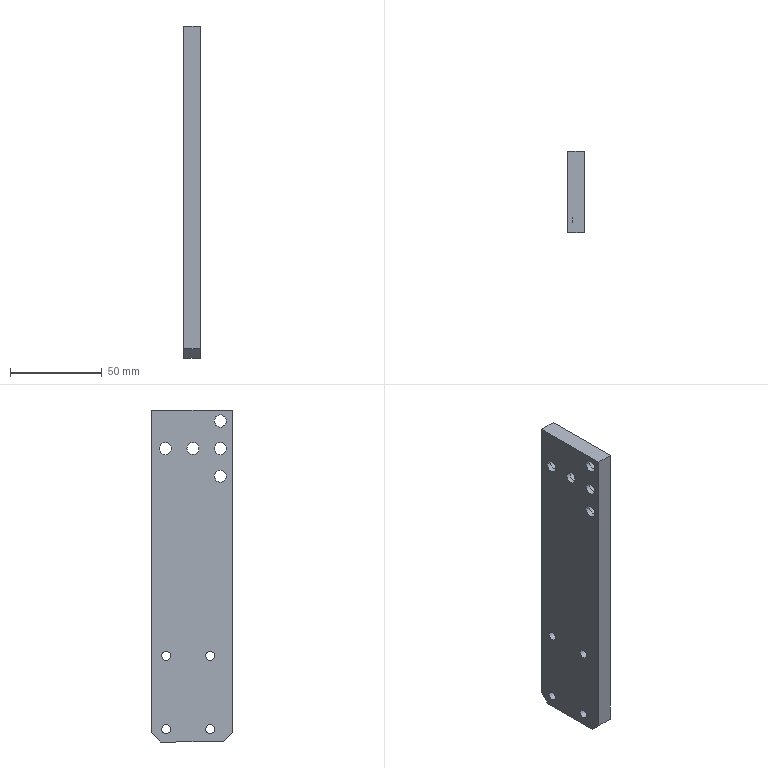Component | SolidWorks | 17081801-804-025A-1 | 1 solid | 41 faces | box 9 x 44 x 181 mm | volume 67258 mm3 | cylinder 28 | plane 13 | commonest cylinder face diameters 11 x10 6.6 x10 5 x8 | material AL6061
build123d program:
from build123d import *

# Parameters (mm, degrees)
SKETCH1_W                                       = 181
SKETCH1_H                                       = 44
BOSS_EXTRUDE1_DEPTH                             = 4.5
M6_TAPPED_HOLE1_D                               = 5
M6_TAPPED_HOLE1_DEPTH                           = 15
M6_TAPPED_HOLE1_TIP                             = 1.502
CHAMFER1_SIZE                                   = 5
M6_HEX_SOCKET_HEAD_CAP_SCREW_CBORE1_D           = 6.6
M6_HEX_SOCKET_HEAD_CAP_SCREW_CBORE1_DEPTH       = 15
M6_HEX_SOCKET_HEAD_CAP_SCREW_CBORE1_CBORE_D     = 11
M6_HEX_SOCKET_HEAD_CAP_SCREW_CBORE1_CBORE_DEPTH = 6.4
M6_HEX_SOCKET_HEAD_CAP_SCREW_CBORE1_TIP         = 1.983
M6_HEX_SOCKET_HEAD_CAP_SCREW_CBORE2_D           = 6.6
M6_HEX_SOCKET_HEAD_CAP_SCREW_CBORE2_DEPTH       = 15
M6_HEX_SOCKET_HEAD_CAP_SCREW_CBORE2_CBORE_D     = 11
M6_HEX_SOCKET_HEAD_CAP_SCREW_CBORE2_CBORE_DEPTH = 6.4
M6_HEX_SOCKET_HEAD_CAP_SCREW_CBORE2_TIP         = 1.983


with BuildPart() as part:
    # Sketch1 → Boss-Extrude1 (new, symmetric)
    with BuildSketch(Plane(origin=(0, 0, 0), x_dir=(1, 0, 0), z_dir=(0, 1, 0))):
        Rectangle(SKETCH1_W, SKETCH1_H)
    extrude(amount=BOSS_EXTRUDE1_DEPTH, both=True)

    # M6 Tapped Hole1
    with Locations(Plane(origin=(0, 4.5, 0), x_dir=(1, 0, 0), z_dir=(0, 1, 0))):
        with Locations((43.5, 10), (83.5, 10), (83.5, -14), (43.5, -14)):
            Hole(M6_TAPPED_HOLE1_D / 2, depth=M6_TAPPED_HOLE1_DEPTH)
            with Locations((0, 0, -(M6_TAPPED_HOLE1_DEPTH + M6_TAPPED_HOLE1_TIP / 2))):  # 118° drill point
                Cone(0, M6_TAPPED_HOLE1_D / 2, M6_TAPPED_HOLE1_TIP, mode=Mode.SUBTRACT)

    # Chamfer1
    chamfer1_edges = [part.edges().sort_by_distance(p)[0] for p in [
        (90.5, 0, -22),
        (90.5, 0, 22),
    ]]
    chamfer(chamfer1_edges, length=CHAMFER1_SIZE)

    # M6 Hex Socket Head Cap Screw CBORE1
    with Locations(Plane.XZ.offset(4.5)):
        with Locations((-84.5, -15.5), (-69.5, -15.5), (-54.5, -15.5)):
            CounterBoreHole(M6_HEX_SOCKET_HEAD_CAP_SCREW_CBORE1_D / 2, M6_HEX_SOCKET_HEAD_CAP_SCREW_CBORE1_CBORE_D / 2, M6_HEX_SOCKET_HEAD_CAP_SCREW_CBORE1_CBORE_DEPTH, depth=M6_HEX_SOCKET_HEAD_CAP_SCREW_CBORE1_DEPTH)
            with Locations((0, 0, -(M6_HEX_SOCKET_HEAD_CAP_SCREW_CBORE1_DEPTH + M6_HEX_SOCKET_HEAD_CAP_SCREW_CBORE1_TIP / 2))):  # 118° drill point
                Cone(0, M6_HEX_SOCKET_HEAD_CAP_SCREW_CBORE1_D / 2, M6_HEX_SOCKET_HEAD_CAP_SCREW_CBORE1_TIP, mode=Mode.SUBTRACT)

    # M6 Hex Socket Head Cap Screw CBORE2
    with Locations(Plane(origin=(0, -4.5, 0), x_dir=(-1, 0, 0), z_dir=(0, -1, 0))):
        with Locations((69.5, 0.5), (69.5, -14.5)):
            CounterBoreHole(M6_HEX_SOCKET_HEAD_CAP_SCREW_CBORE2_D / 2, M6_HEX_SOCKET_HEAD_CAP_SCREW_CBORE2_CBORE_D / 2, M6_HEX_SOCKET_HEAD_CAP_SCREW_CBORE2_CBORE_DEPTH, depth=M6_HEX_SOCKET_HEAD_CAP_SCREW_CBORE2_DEPTH)
            with Locations((0, 0, -(M6_HEX_SOCKET_HEAD_CAP_SCREW_CBORE2_DEPTH + M6_HEX_SOCKET_HEAD_CAP_SCREW_CBORE2_TIP / 2))):  # 118° drill point
                Cone(0, M6_HEX_SOCKET_HEAD_CAP_SCREW_CBORE2_D / 2, M6_HEX_SOCKET_HEAD_CAP_SCREW_CBORE2_TIP, mode=Mode.SUBTRACT)


solid = part.part

# Placed as in the assembly
solid = solid.moved(Location((241.5, 2120.9, 101.5), (-90, 0, 90)))